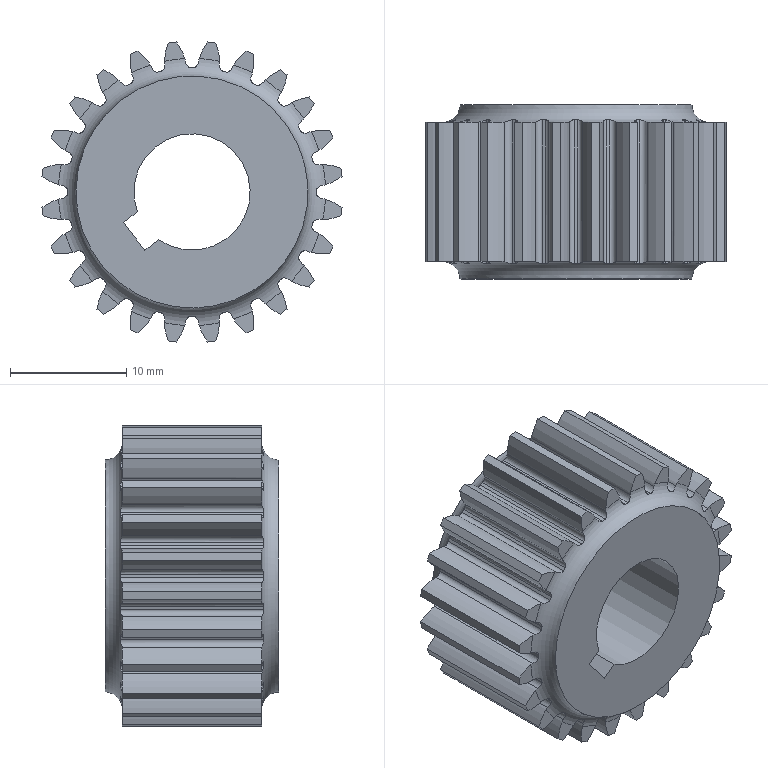Component | NX | SMALL_GEAR | 1 solid | 200 faces | volume 5091 mm3 | spline 120 | plane 53 | cylinder 25 | torus 2 | commonest cylinder face diameters 21.48 x24 10.02 x1